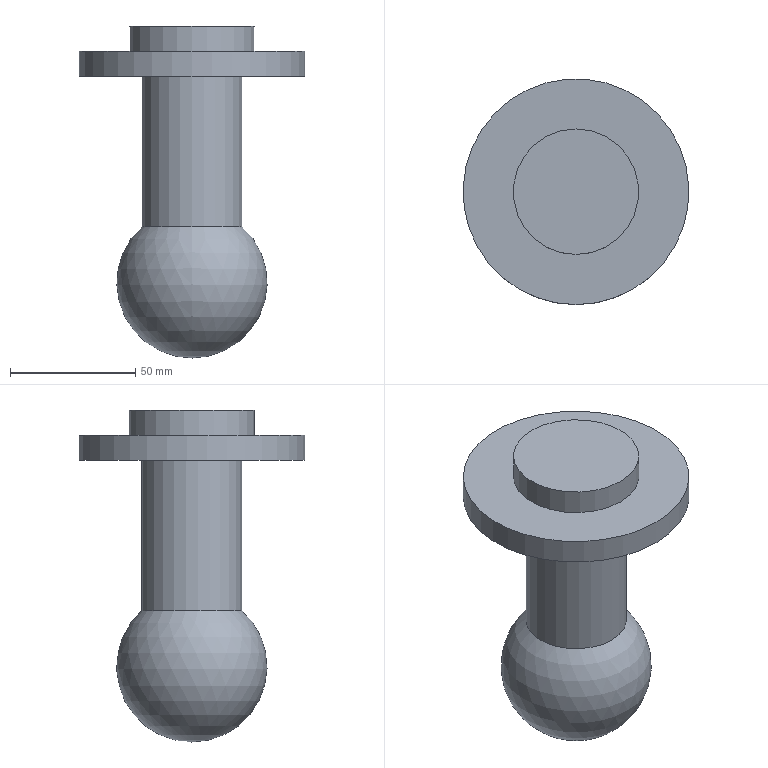Component | NX | BALL_MOUNT | 1 solid | 7 faces | box 90 x 90 x 132.36 mm | volume 266714 mm3 | cylinder 3 | plane 3 | sphere 1 | commonest cylinder face diameters 40 x1 90 x1 50 x1
STEP:
#1=CARTESIAN_POINT('',(0.,0.,0.));
#2=DIRECTION('',(0.,0.,1.));
#3=DIRECTION('',(1.,0.,0.));
#4=AXIS2_PLACEMENT_3D('',#1,#2,#3);
#5=CARTESIAN_POINT('',(562.45,-20.,245.361));
#6=VERTEX_POINT('',#5);
#7=CARTESIAN_POINT('',(562.45,0.,245.361));
#8=DIRECTION('',(0.,-0.,1.));
#9=DIRECTION('',(0.,-1.,-0.));
#10=AXIS2_PLACEMENT_3D('',#7,#8,#9);
#11=CIRCLE('',#10,20.);
#12=CARTESIAN_POINT('',(562.45,0.,223.));
#13=DIRECTION('',(0.,-0.,1.));
#14=DIRECTION('',(0.,-1.,-0.));
#15=AXIS2_PLACEMENT_3D('',#12,#13,#14);
#16=SPHERICAL_SURFACE('',#15,30.);
#17=CARTESIAN_POINT('',(0.,0.8411));
#18=CARTESIAN_POINT('',(0.0952,0.8411));
#19=CARTESIAN_POINT('',(0.2856,0.8411));
#20=CARTESIAN_POINT('',(0.5712,0.8411));
#21=CARTESIAN_POINT('',(0.8568,0.8411));
#22=CARTESIAN_POINT('',(1.142,0.8411));
#23=CARTESIAN_POINT('',(1.428,0.8411));
#24=CARTESIAN_POINT('',(1.714,0.8411));
#25=CARTESIAN_POINT('',(1.999,0.8411));
#26=CARTESIAN_POINT('',(2.285,0.8411));
#27=CARTESIAN_POINT('',(2.57,0.8411));
#28=CARTESIAN_POINT('',(2.856,0.8411));
#29=CARTESIAN_POINT('',(3.142,0.8411));
#30=CARTESIAN_POINT('',(3.427,0.8411));
#31=CARTESIAN_POINT('',(3.713,0.8411));
#32=CARTESIAN_POINT('',(3.998,0.8411));
#33=CARTESIAN_POINT('',(4.284,0.8411));
#34=CARTESIAN_POINT('',(4.57,0.8411));
#35=CARTESIAN_POINT('',(4.855,0.8411));
#36=CARTESIAN_POINT('',(5.141,0.8411));
#37=CARTESIAN_POINT('',(5.426,0.8411));
#38=CARTESIAN_POINT('',(5.712,0.8411));
#39=CARTESIAN_POINT('',(5.998,0.8411));
#40=CARTESIAN_POINT('',(6.188,0.8411));
#41=CARTESIAN_POINT('',(6.283,0.8411));
#42=B_SPLINE_CURVE_WITH_KNOTS('',3,(#17,#18,#19,#20,#21,#22,#23,#24,#25,#26,#27,#28,#29,#30,#31,#32,#33,#34,#35,#36,#37,#38,#39,#40,#41),.UNSPECIFIED.,.F.,.F.,(4,1,1,1,1,1,1,1,1,1,1,1,1,1,1,1,1,1,1,1,1,1,4),(0.,0.2856,0.5712,0.8568,1.142,1.428,1.714,1.999,2.285,2.57,2.856,3.142,3.427,3.713,3.998,4.284,4.57,4.855,5.141,5.426,5.712,5.998,6.283),.QUASI_UNIFORM_KNOTS.);
#43=(GEOMETRIC_REPRESENTATION_CONTEXT(2)PARAMETRIC_REPRESENTATION_CONTEXT()REPRESENTATION_CONTEXT('',''));
#44=DEFINITIONAL_REPRESENTATION('',(#42),#43);
#45=PCURVE('',#16,#44);
#46=CARTESIAN_POINT('',(562.45,-0.,390.361));
#47=DIRECTION('',(0.,-0.,1.));
#48=DIRECTION('',(0.,-1.,-0.));
#49=AXIS2_PLACEMENT_3D('',#46,#47,#48);
#50=CYLINDRICAL_SURFACE('',#49,20.);
#51=CARTESIAN_POINT('',(0.,-145.));
#52=DIRECTION('',(1.,0.));
#53=VECTOR('',#52,1.);
#54=LINE('',#51,#53);
#55=(GEOMETRIC_REPRESENTATION_CONTEXT(2)PARAMETRIC_REPRESENTATION_CONTEXT()REPRESENTATION_CONTEXT('',''));
#56=DEFINITIONAL_REPRESENTATION('',(#54),#55);
#57=PCURVE('',#50,#56);
#58=SURFACE_CURVE('',#11,(#45,#57),.PCURVE_S1.);
#59=EDGE_CURVE('',#6,#6,#58,.T.);
#60=ORIENTED_EDGE('',*,*,#59,.F.);
#61=CARTESIAN_POINT('',(562.45,0.,193.));
#62=VERTEX_POINT('',#61);
#63=CARTESIAN_POINT('',(562.45,0.,193.));
#64=CARTESIAN_POINT('',(562.45,-9.044,193.));
#65=CARTESIAN_POINT('',(562.45,-18.089,196.116));
#66=CARTESIAN_POINT('',(562.45,-25.881,202.348));
#67=CARTESIAN_POINT('',(562.45,-31.168,211.095));
#68=CARTESIAN_POINT('',(562.45,-33.058,221.139));
#69=CARTESIAN_POINT('',(562.45,-31.405,230.978));
#70=CARTESIAN_POINT('',(562.45,-26.741,239.331));
#71=CARTESIAN_POINT('',(562.45,-20.,245.361));
#72=B_SPLINE_CURVE_WITH_KNOTS('',8,(#63,#64,#65,#66,#67,#68,#69,#70,#71),.UNSPECIFIED.,.F.,.F.,(9,9),(-1.571,0.8411),.PIECEWISE_BEZIER_KNOTS.);
#73=CARTESIAN_POINT('',(0.,0.));
#74=DIRECTION('',(0.,1.));
#75=VECTOR('',#74,1.);
#76=LINE('',#73,#75);
#77=(GEOMETRIC_REPRESENTATION_CONTEXT(2)PARAMETRIC_REPRESENTATION_CONTEXT()REPRESENTATION_CONTEXT('',''));
#78=DEFINITIONAL_REPRESENTATION('',(#76),#77);
#79=PCURVE('',#16,#78);
#80=CARTESIAN_POINT('',(6.283,0.));
#81=DIRECTION('',(0.,1.));
#82=VECTOR('',#81,1.);
#83=LINE('',#80,#82);
#84=(GEOMETRIC_REPRESENTATION_CONTEXT(2)PARAMETRIC_REPRESENTATION_CONTEXT()REPRESENTATION_CONTEXT('',''));
#85=DEFINITIONAL_REPRESENTATION('',(#83),#84);
#86=PCURVE('',#16,#85);
#87=SEAM_CURVE('',#72,(#79,#86),.PCURVE_S1.);
#88=EDGE_CURVE('',#62,#6,#87,.T.);
#89=ORIENTED_EDGE('',*,*,#88,.F.);
#90=ORIENTED_EDGE('',*,*,#88,.T.);
#91=EDGE_LOOP('',(#60,#89,#90));
#92=FACE_BOUND('',#91,.T.);
#93=ADVANCED_FACE('',(#92),#16,.T.);
#94=ORIENTED_EDGE('',*,*,#59,.T.);
#95=CARTESIAN_POINT('',(562.45,-20.,305.361));
#96=VERTEX_POINT('',#95);
#97=CARTESIAN_POINT('',(562.45,-20.,245.361));
#98=CARTESIAN_POINT('',(562.45,-20.,305.361));
#99=B_SPLINE_CURVE_WITH_KNOTS('',1,(#97,#98),.UNSPECIFIED.,.F.,.F.,(2,2),(-145.,-85.),.PIECEWISE_BEZIER_KNOTS.);
#100=CARTESIAN_POINT('',(6.283,0.));
#101=DIRECTION('',(0.,1.));
#102=VECTOR('',#101,1.);
#103=LINE('',#100,#102);
#104=(GEOMETRIC_REPRESENTATION_CONTEXT(2)PARAMETRIC_REPRESENTATION_CONTEXT()REPRESENTATION_CONTEXT('',''));
#105=DEFINITIONAL_REPRESENTATION('',(#103),#104);
#106=PCURVE('',#50,#105);
#107=CARTESIAN_POINT('',(0.,0.));
#108=DIRECTION('',(0.,1.));
#109=VECTOR('',#108,1.);
#110=LINE('',#107,#109);
#111=(GEOMETRIC_REPRESENTATION_CONTEXT(2)PARAMETRIC_REPRESENTATION_CONTEXT()REPRESENTATION_CONTEXT('',''));
#112=DEFINITIONAL_REPRESENTATION('',(#110),#111);
#113=PCURVE('',#50,#112);
#114=SEAM_CURVE('',#99,(#106,#113),.PCURVE_S1.);
#115=EDGE_CURVE('',#6,#96,#114,.T.);
#116=ORIENTED_EDGE('',*,*,#115,.T.);
#117=CARTESIAN_POINT('',(562.45,-0.,305.361));
#118=DIRECTION('',(0.,-0.,1.));
#119=DIRECTION('',(0.,-1.,-0.));
#120=AXIS2_PLACEMENT_3D('',#117,#118,#119);
#121=CIRCLE('',#120,20.);
#122=CARTESIAN_POINT('',(0.,-85.));
#123=DIRECTION('',(1.,0.));
#124=VECTOR('',#123,1.);
#125=LINE('',#122,#124);
#126=(GEOMETRIC_REPRESENTATION_CONTEXT(2)PARAMETRIC_REPRESENTATION_CONTEXT()REPRESENTATION_CONTEXT('',''));
#127=DEFINITIONAL_REPRESENTATION('',(#125),#126);
#128=PCURVE('',#50,#127);
#129=CARTESIAN_POINT('',(562.45,-45.,305.361));
#130=DIRECTION('',(0.,0.,-1.));
#131=DIRECTION('',(0.,1.,0.));
#132=AXIS2_PLACEMENT_3D('',#129,#130,#131);
#133=PLANE('',#132);
#134=CARTESIAN_POINT('',(25.,0.));
#135=CARTESIAN_POINT('',(25.,34.641));
#136=CARTESIAN_POINT('',(55.,17.321));
#137=CARTESIAN_POINT('',(85.,0.));
#138=CARTESIAN_POINT('',(55.,-17.321));
#139=CARTESIAN_POINT('',(25.,-34.641));
#140=CARTESIAN_POINT('',(25.,0.));
#141=(BOUNDED_CURVE()B_SPLINE_CURVE(2,(#134,#135,#136,#137,#138,#139,#140),.UNSPECIFIED.,.T.,.F.)B_SPLINE_CURVE_WITH_KNOTS((1,2,2,2,2,1),(-2.094,0.,2.094,4.189,6.283,8.378),.UNSPECIFIED.)CURVE()GEOMETRIC_REPRESENTATION_ITEM()RATIONAL_B_SPLINE_CURVE((1.,0.5,1.,0.5,1.,0.5,1.))REPRESENTATION_ITEM(''));
#142=(GEOMETRIC_REPRESENTATION_CONTEXT(2)PARAMETRIC_REPRESENTATION_CONTEXT()REPRESENTATION_CONTEXT('',''));
#143=DEFINITIONAL_REPRESENTATION('',(#141),#142);
#144=PCURVE('',#133,#143);
#145=SURFACE_CURVE('',#121,(#128,#144),.PCURVE_S1.);
#146=EDGE_CURVE('',#96,#96,#145,.T.);
#147=ORIENTED_EDGE('',*,*,#146,.F.);
#148=ORIENTED_EDGE('',*,*,#115,.F.);
#149=EDGE_LOOP('',(#94,#116,#147,#148));
#150=FACE_BOUND('',#149,.T.);
#151=ADVANCED_FACE('',(#150),#50,.T.);
#152=ORIENTED_EDGE('',*,*,#146,.T.);
#153=EDGE_LOOP('',(#152));
#154=FACE_BOUND('',#153,.T.);
#155=CARTESIAN_POINT('',(562.45,-45.,305.361));
#156=VERTEX_POINT('',#155);
#157=CARTESIAN_POINT('',(562.45,-0.,305.361));
#158=DIRECTION('',(0.,-0.,1.));
#159=DIRECTION('',(0.,-1.,-0.));
#160=AXIS2_PLACEMENT_3D('',#157,#158,#159);
#161=CIRCLE('',#160,45.);
#162=CARTESIAN_POINT('',(-0.,0.));
#163=CARTESIAN_POINT('',(-0.,77.942));
#164=CARTESIAN_POINT('',(67.5,38.971));
#165=CARTESIAN_POINT('',(135.,0.));
#166=CARTESIAN_POINT('',(67.5,-38.971));
#167=CARTESIAN_POINT('',(0.,-77.942));
#168=CARTESIAN_POINT('',(-0.,0.));
#169=(BOUNDED_CURVE()B_SPLINE_CURVE(2,(#162,#163,#164,#165,#166,#167,#168),.UNSPECIFIED.,.T.,.F.)B_SPLINE_CURVE_WITH_KNOTS((1,2,2,2,2,1),(-2.094,0.,2.094,4.189,6.283,8.378),.UNSPECIFIED.)CURVE()GEOMETRIC_REPRESENTATION_ITEM()RATIONAL_B_SPLINE_CURVE((1.,0.5,1.,0.5,1.,0.5,1.))REPRESENTATION_ITEM(''));
#170=(GEOMETRIC_REPRESENTATION_CONTEXT(2)PARAMETRIC_REPRESENTATION_CONTEXT()REPRESENTATION_CONTEXT('',''));
#171=DEFINITIONAL_REPRESENTATION('',(#169),#170);
#172=PCURVE('',#133,#171);
#173=CARTESIAN_POINT('',(562.45,-0.,390.361));
#174=DIRECTION('',(0.,-0.,1.));
#175=DIRECTION('',(0.,-1.,-0.));
#176=AXIS2_PLACEMENT_3D('',#173,#174,#175);
#177=CYLINDRICAL_SURFACE('',#176,45.);
#178=CARTESIAN_POINT('',(0.,-85.));
#179=DIRECTION('',(1.,0.));
#180=VECTOR('',#179,1.);
#181=LINE('',#178,#180);
#182=(GEOMETRIC_REPRESENTATION_CONTEXT(2)PARAMETRIC_REPRESENTATION_CONTEXT()REPRESENTATION_CONTEXT('',''));
#183=DEFINITIONAL_REPRESENTATION('',(#181),#182);
#184=PCURVE('',#177,#183);
#185=SURFACE_CURVE('',#161,(#172,#184),.PCURVE_S1.);
#186=EDGE_CURVE('',#156,#156,#185,.T.);
#187=ORIENTED_EDGE('',*,*,#186,.F.);
#188=EDGE_LOOP('',(#187));
#189=FACE_BOUND('',#188,.T.);
#190=ADVANCED_FACE('',(#154,#189),#133,.T.);
#191=ORIENTED_EDGE('',*,*,#186,.T.);
#192=CARTESIAN_POINT('',(562.45,-45.,315.361));
#193=VERTEX_POINT('',#192);
#194=CARTESIAN_POINT('',(562.45,-45.,305.361));
#195=CARTESIAN_POINT('',(562.45,-45.,315.361));
#196=B_SPLINE_CURVE_WITH_KNOTS('',1,(#194,#195),.UNSPECIFIED.,.F.,.F.,(2,2),(-85.,-75.),.PIECEWISE_BEZIER_KNOTS.);
#197=CARTESIAN_POINT('',(6.283,0.));
#198=DIRECTION('',(0.,1.));
#199=VECTOR('',#198,1.);
#200=LINE('',#197,#199);
#201=(GEOMETRIC_REPRESENTATION_CONTEXT(2)PARAMETRIC_REPRESENTATION_CONTEXT()REPRESENTATION_CONTEXT('',''));
#202=DEFINITIONAL_REPRESENTATION('',(#200),#201);
#203=PCURVE('',#177,#202);
#204=CARTESIAN_POINT('',(0.,0.));
#205=DIRECTION('',(0.,1.));
#206=VECTOR('',#205,1.);
#207=LINE('',#204,#206);
#208=(GEOMETRIC_REPRESENTATION_CONTEXT(2)PARAMETRIC_REPRESENTATION_CONTEXT()REPRESENTATION_CONTEXT('',''));
#209=DEFINITIONAL_REPRESENTATION('',(#207),#208);
#210=PCURVE('',#177,#209);
#211=SEAM_CURVE('',#196,(#203,#210),.PCURVE_S1.);
#212=EDGE_CURVE('',#156,#193,#211,.T.);
#213=ORIENTED_EDGE('',*,*,#212,.T.);
#214=CARTESIAN_POINT('',(562.45,-0.,315.361));
#215=DIRECTION('',(0.,-0.,1.));
#216=DIRECTION('',(0.,-1.,-0.));
#217=AXIS2_PLACEMENT_3D('',#214,#215,#216);
#218=CIRCLE('',#217,45.);
#219=CARTESIAN_POINT('',(0.,-75.));
#220=DIRECTION('',(1.,0.));
#221=VECTOR('',#220,1.);
#222=LINE('',#219,#221);
#223=(GEOMETRIC_REPRESENTATION_CONTEXT(2)PARAMETRIC_REPRESENTATION_CONTEXT()REPRESENTATION_CONTEXT('',''));
#224=DEFINITIONAL_REPRESENTATION('',(#222),#223);
#225=PCURVE('',#177,#224);
#226=CARTESIAN_POINT('',(562.45,-25.,315.361));
#227=DIRECTION('',(0.,-0.,1.));
#228=DIRECTION('',(0.,-1.,-0.));
#229=AXIS2_PLACEMENT_3D('',#226,#227,#228);
#230=PLANE('',#229);
#231=CARTESIAN_POINT('',(-25.,0.));
#232=DIRECTION('',(1.,0.));
#233=AXIS2_PLACEMENT_2D('',#231,#232);
#234=CIRCLE('',#233,45.);
#235=(GEOMETRIC_REPRESENTATION_CONTEXT(2)PARAMETRIC_REPRESENTATION_CONTEXT()REPRESENTATION_CONTEXT('',''));
#236=DEFINITIONAL_REPRESENTATION('',(#234),#235);
#237=PCURVE('',#230,#236);
#238=SURFACE_CURVE('',#218,(#225,#237),.PCURVE_S1.);
#239=EDGE_CURVE('',#193,#193,#238,.T.);
#240=ORIENTED_EDGE('',*,*,#239,.F.);
#241=ORIENTED_EDGE('',*,*,#212,.F.);
#242=EDGE_LOOP('',(#191,#213,#240,#241));
#243=FACE_BOUND('',#242,.T.);
#244=ADVANCED_FACE('',(#243),#177,.T.);
#245=ORIENTED_EDGE('',*,*,#239,.T.);
#246=EDGE_LOOP('',(#245));
#247=FACE_BOUND('',#246,.T.);
#248=CARTESIAN_POINT('',(562.45,-25.,315.361));
#249=VERTEX_POINT('',#248);
#250=CARTESIAN_POINT('',(562.45,-0.,315.361));
#251=DIRECTION('',(0.,-0.,1.));
#252=DIRECTION('',(0.,-1.,-0.));
#253=AXIS2_PLACEMENT_3D('',#250,#251,#252);
#254=CIRCLE('',#253,25.);
#255=CARTESIAN_POINT('',(-25.,0.));
#256=DIRECTION('',(1.,0.));
#257=AXIS2_PLACEMENT_2D('',#255,#256);
#258=CIRCLE('',#257,25.);
#259=(GEOMETRIC_REPRESENTATION_CONTEXT(2)PARAMETRIC_REPRESENTATION_CONTEXT()REPRESENTATION_CONTEXT('',''));
#260=DEFINITIONAL_REPRESENTATION('',(#258),#259);
#261=PCURVE('',#230,#260);
#262=CARTESIAN_POINT('',(562.45,-0.,390.361));
#263=DIRECTION('',(0.,-0.,1.));
#264=DIRECTION('',(0.,-1.,-0.));
#265=AXIS2_PLACEMENT_3D('',#262,#263,#264);
#266=CYLINDRICAL_SURFACE('',#265,25.);
#267=CARTESIAN_POINT('',(0.,-75.));
#268=DIRECTION('',(1.,0.));
#269=VECTOR('',#268,1.);
#270=LINE('',#267,#269);
#271=(GEOMETRIC_REPRESENTATION_CONTEXT(2)PARAMETRIC_REPRESENTATION_CONTEXT()REPRESENTATION_CONTEXT('',''));
#272=DEFINITIONAL_REPRESENTATION('',(#270),#271);
#273=PCURVE('',#266,#272);
#274=SURFACE_CURVE('',#254,(#261,#273),.PCURVE_S1.);
#275=EDGE_CURVE('',#249,#249,#274,.T.);
#276=ORIENTED_EDGE('',*,*,#275,.F.);
#277=EDGE_LOOP('',(#276));
#278=FACE_BOUND('',#277,.T.);
#279=ADVANCED_FACE('',(#247,#278),#230,.T.);
#280=ORIENTED_EDGE('',*,*,#275,.T.);
#281=CARTESIAN_POINT('',(562.45,-25.,325.361));
#282=VERTEX_POINT('',#281);
#283=CARTESIAN_POINT('',(562.45,-25.,315.361));
#284=CARTESIAN_POINT('',(562.45,-25.,325.361));
#285=B_SPLINE_CURVE_WITH_KNOTS('',1,(#283,#284),.UNSPECIFIED.,.F.,.F.,(2,2),(-75.,-65.),.PIECEWISE_BEZIER_KNOTS.);
#286=CARTESIAN_POINT('',(6.283,0.));
#287=DIRECTION('',(0.,1.));
#288=VECTOR('',#287,1.);
#289=LINE('',#286,#288);
#290=(GEOMETRIC_REPRESENTATION_CONTEXT(2)PARAMETRIC_REPRESENTATION_CONTEXT()REPRESENTATION_CONTEXT('',''));
#291=DEFINITIONAL_REPRESENTATION('',(#289),#290);
#292=PCURVE('',#266,#291);
#293=CARTESIAN_POINT('',(0.,0.));
#294=DIRECTION('',(0.,1.));
#295=VECTOR('',#294,1.);
#296=LINE('',#293,#295);
#297=(GEOMETRIC_REPRESENTATION_CONTEXT(2)PARAMETRIC_REPRESENTATION_CONTEXT()REPRESENTATION_CONTEXT('',''));
#298=DEFINITIONAL_REPRESENTATION('',(#296),#297);
#299=PCURVE('',#266,#298);
#300=SEAM_CURVE('',#285,(#292,#299),.PCURVE_S1.);
#301=EDGE_CURVE('',#249,#282,#300,.T.);
#302=ORIENTED_EDGE('',*,*,#301,.T.);
#303=CARTESIAN_POINT('',(562.45,-0.,325.361));
#304=DIRECTION('',(0.,-0.,1.));
#305=DIRECTION('',(0.,-1.,-0.));
#306=AXIS2_PLACEMENT_3D('',#303,#304,#305);
#307=CIRCLE('',#306,25.);
#308=CARTESIAN_POINT('',(0.,-65.));
#309=DIRECTION('',(1.,0.));
#310=VECTOR('',#309,1.);
#311=LINE('',#308,#310);
#312=(GEOMETRIC_REPRESENTATION_CONTEXT(2)PARAMETRIC_REPRESENTATION_CONTEXT()REPRESENTATION_CONTEXT('',''));
#313=DEFINITIONAL_REPRESENTATION('',(#311),#312);
#314=PCURVE('',#266,#313);
#315=CARTESIAN_POINT('',(562.45,-0.,325.361));
#316=DIRECTION('',(0.,-0.,1.));
#317=DIRECTION('',(0.,-1.,-0.));
#318=AXIS2_PLACEMENT_3D('',#315,#316,#317);
#319=PLANE('',#318);
#320=CARTESIAN_POINT('',(0.,0.));
#321=DIRECTION('',(1.,0.));
#322=AXIS2_PLACEMENT_2D('',#320,#321);
#323=CIRCLE('',#322,25.);
#324=(GEOMETRIC_REPRESENTATION_CONTEXT(2)PARAMETRIC_REPRESENTATION_CONTEXT()REPRESENTATION_CONTEXT('',''));
#325=DEFINITIONAL_REPRESENTATION('',(#323),#324);
#326=PCURVE('',#319,#325);
#327=SURFACE_CURVE('',#307,(#314,#326),.PCURVE_S1.);
#328=EDGE_CURVE('',#282,#282,#327,.T.);
#329=ORIENTED_EDGE('',*,*,#328,.F.);
#330=ORIENTED_EDGE('',*,*,#301,.F.);
#331=EDGE_LOOP('',(#280,#302,#329,#330));
#332=FACE_BOUND('',#331,.T.);
#333=ADVANCED_FACE('',(#332),#266,.T.);
#334=ORIENTED_EDGE('',*,*,#328,.T.);
#335=EDGE_LOOP('',(#334));
#336=FACE_BOUND('',#335,.T.);
#337=ADVANCED_FACE('',(#336),#319,.T.);
#338=CLOSED_SHELL('',(#93,#151,#190,#244,#279,#333,#337));
#339=MANIFOLD_SOLID_BREP('',#338);
#340=(LENGTH_UNIT()NAMED_UNIT(*)SI_UNIT(.MILLI.,.METRE.));
#341=UNCERTAINTY_MEASURE_WITH_UNIT(LENGTH_MEASURE(0.00001),#340,'','');
#342=(NAMED_UNIT(*)PLANE_ANGLE_UNIT()SI_UNIT($,.RADIAN.));
#343=(NAMED_UNIT(*)SI_UNIT($,.STERADIAN.)SOLID_ANGLE_UNIT());
#344=(GEOMETRIC_REPRESENTATION_CONTEXT(3)GLOBAL_UNCERTAINTY_ASSIGNED_CONTEXT((#341))GLOBAL_UNIT_ASSIGNED_CONTEXT((#340,#342,#343))REPRESENTATION_CONTEXT('',''));
#345=ADVANCED_BREP_SHAPE_REPRESENTATION('',(#4,#339),#344);